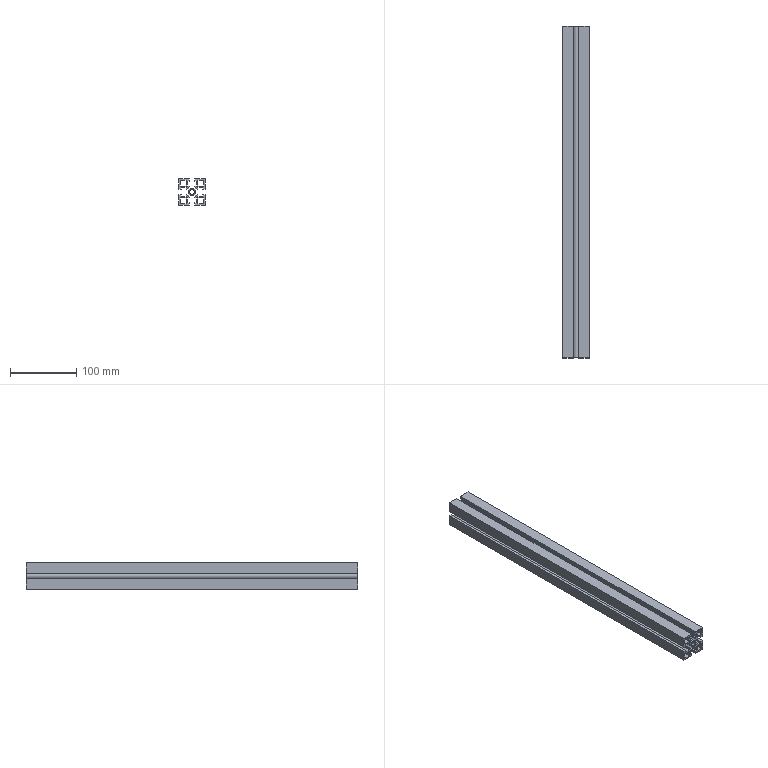Component | SolidWorks | AluminumProfile500-1 | 1 solid | 89 faces | box 40 x 500 x 40 mm | volume 290037 mm3 | plane 82 | cylinder 7 | commonest cylinder face diameters 10.5 x5 6.8 x2 | material 6061 Alloy
build123d program:
from build123d import *

# Parameters (mm, degrees)
SKETCH1_W                  = 40
SKETCH1_H                  = 40
EXTRUDE1_DEPTH             = 1640
CUT_EXTRUDE1_DEPTH         = 1641.975
SKETCH3_R                  = 3.4
CUT_EXTRUDE2_DEPTH         = 1641.975
CIRPATTERN1_COUNT          = 4
EXTRUDE2_DEPTH             = 1641.975
CIRPATTERN2_COUNT          = 4
SKETCH5_W                  = 9
SKETCH5_H                  = 9
EXTRUDE3_DEPTH             = 1641.975
CIRPATTERN3_COUNT          = 4
M8X1_25_TAPPED_HOLE3_D     = 6.8
M8X1_25_TAPPED_HOLE3_DEPTH = 19.75
M8X1_25_TAPPED_HOLE3_TIP   = 2.043
SKETCH9_W                  = 177.591
SKETCH9_H                  = 2021.808
CUT_EXTRUDE3_DEPTH         = 1641.975


with BuildPart() as part:
    # Sketch1 → Extrude1 (new body)
    with BuildSketch(Plane.XY):
        with Locations((20, 20)):
            Rectangle(SKETCH1_W, SKETCH1_H)
    extrude(amount=EXTRUDE1_DEPTH)

    # Sketch2 → Cut-Extrude1 (cut, through all)
    with BuildSketch(Plane.XY.offset(1640)):
        Polygon((16, 40), (16, 36), (13, 36), (13, 29), (27, 29), (27, 36), (24, 36), (24, 40), align=None)
    cut_extrude1 = extrude(amount=-CUT_EXTRUDE1_DEPTH, mode=Mode.SUBTRACT)

    # Sketch3 → Cut-Extrude2 (cut, through all)
    with BuildSketch(Plane.XY.offset(1640)):
        with Locations((20, 20)):
            Circle(SKETCH3_R)
    extrude(amount=-CUT_EXTRUDE2_DEPTH, mode=Mode.SUBTRACT)

    # CirPattern1: Cut-Extrude1 ×4 about axis
    cirpattern1_axis = Axis((20, 20, 0), (0, 0, 1))
    for i in range(1, CIRPATTERN1_COUNT):
        add(cut_extrude1.rotate(cirpattern1_axis, i * 360 / CIRPATTERN1_COUNT), mode=Mode.SUBTRACT)

    # Sketch4 → Extrude2 (cut, through all)
    with BuildSketch(Plane.XY.offset(1640)):
        with BuildLine():
            Line((15.75, 29), (16.457, 28.293))
            Line((16.457, 28.293), (14.806, 26.641))
            Line((14.806, 26.641), (17.082, 24.365))
            ThreePointArc((17.082, 24.365), (20, 25.25), (22.918, 24.365))
            Line((22.918, 24.365), (25.194, 26.641))
            Line((25.194, 26.641), (23.543, 28.293))
            Line((23.543, 28.293), (24.25, 29))
            Line((24.25, 29), (15.75, 29))
        make_face()
    extrude2 = extrude(amount=-EXTRUDE2_DEPTH, mode=Mode.SUBTRACT)

    # CirPattern2: Extrude2 ×4 about axis
    cirpattern2_axis = Axis((20, 20, 0), (0, 0, 1))
    for i in range(1, CIRPATTERN2_COUNT):
        add(extrude2.rotate(cirpattern2_axis, i * 360 / CIRPATTERN2_COUNT), mode=Mode.SUBTRACT)

    # Sketch5 → Extrude3 (cut, through all)
    with BuildSketch(Plane.XY.offset(1640)):
        with Locations((6.5, 33.5)):
            Rectangle(SKETCH5_W, SKETCH5_H)
    extrude3 = extrude(amount=-EXTRUDE3_DEPTH, mode=Mode.SUBTRACT)

    # CirPattern3: Extrude3 ×4 about axis
    cirpattern3_axis = Axis((20, 20, 0), (0, 0, 1))
    for i in range(1, CIRPATTERN3_COUNT):
        add(extrude3.rotate(cirpattern3_axis, i * 360 / CIRPATTERN3_COUNT), mode=Mode.SUBTRACT)

    # M8x1.25 Tapped Hole3
    with Locations(Plane(origin=(20, 20, 1640), x_dir=(1, 0, 0), z_dir=(0, 0, 1))):
        with Locations((0, 0)):
            Hole(M8X1_25_TAPPED_HOLE3_D / 2, depth=M8X1_25_TAPPED_HOLE3_DEPTH)
            with Locations((0, 0, -(M8X1_25_TAPPED_HOLE3_DEPTH + M8X1_25_TAPPED_HOLE3_TIP / 2))):  # 118° drill point
                Cone(0, M8X1_25_TAPPED_HOLE3_D / 2, M8X1_25_TAPPED_HOLE3_TIP, mode=Mode.SUBTRACT)

    # Sketch9 → Cut-Extrude3 (cut, through all)
    with BuildSketch(Plane.XZ):
        with Locations((13.869, 1510.904)):
            Rectangle(SKETCH9_W, SKETCH9_H)
    extrude(amount=-CUT_EXTRUDE3_DEPTH, mode=Mode.SUBTRACT)


solid = part.part

# Placed as in the assembly
solid = solid.moved(Location((-1288.352, -468.217, -96.285), (90, 0, 0)))